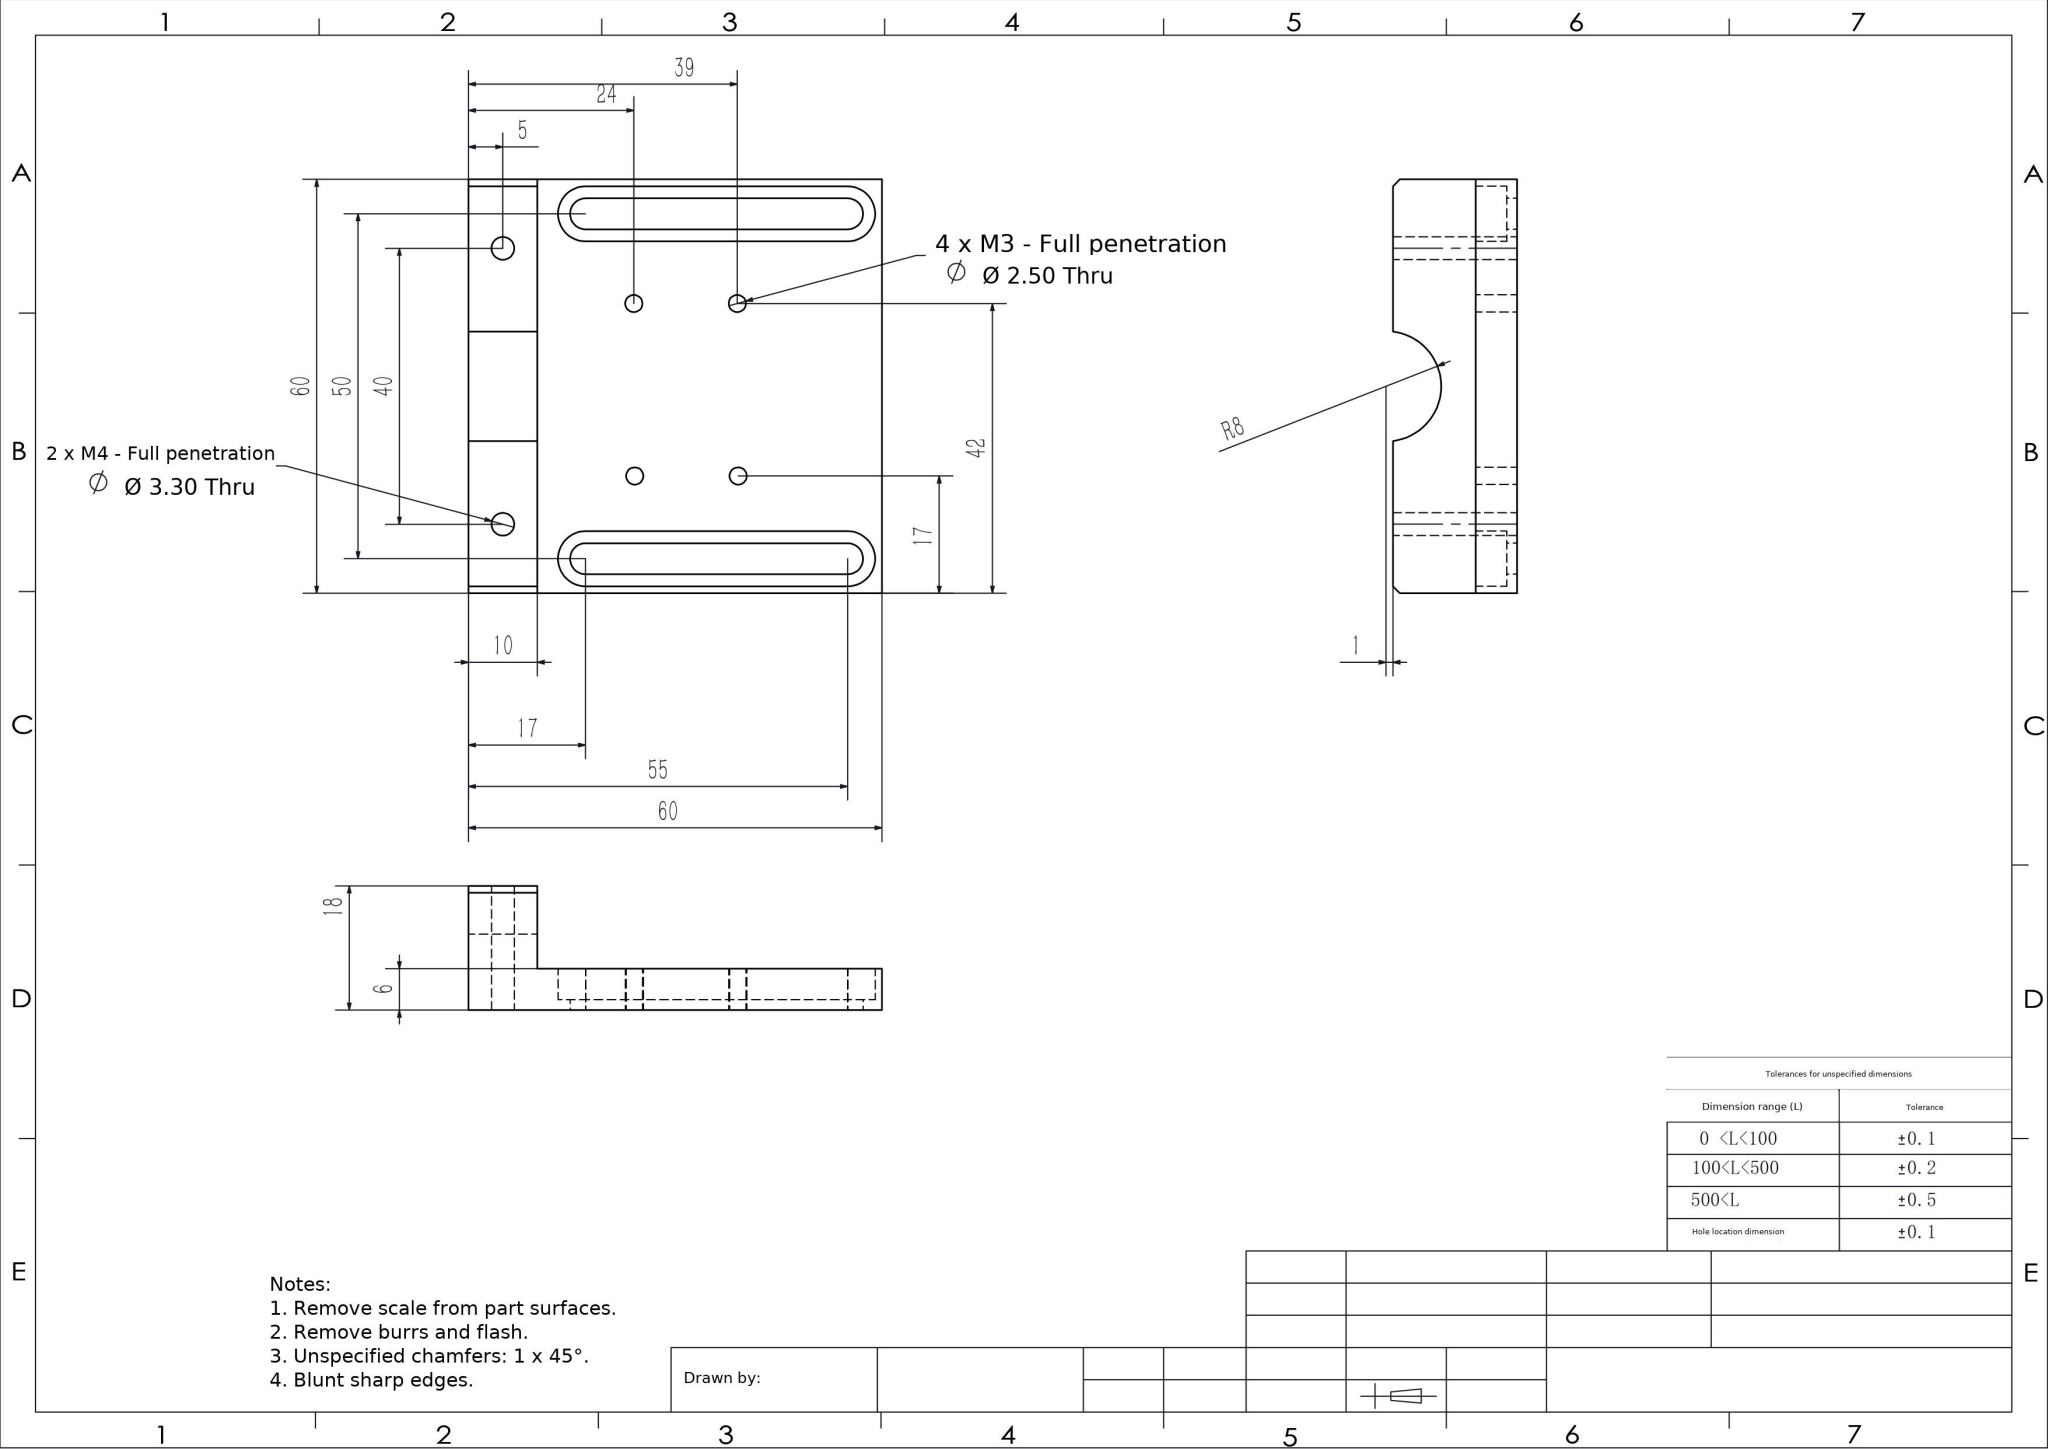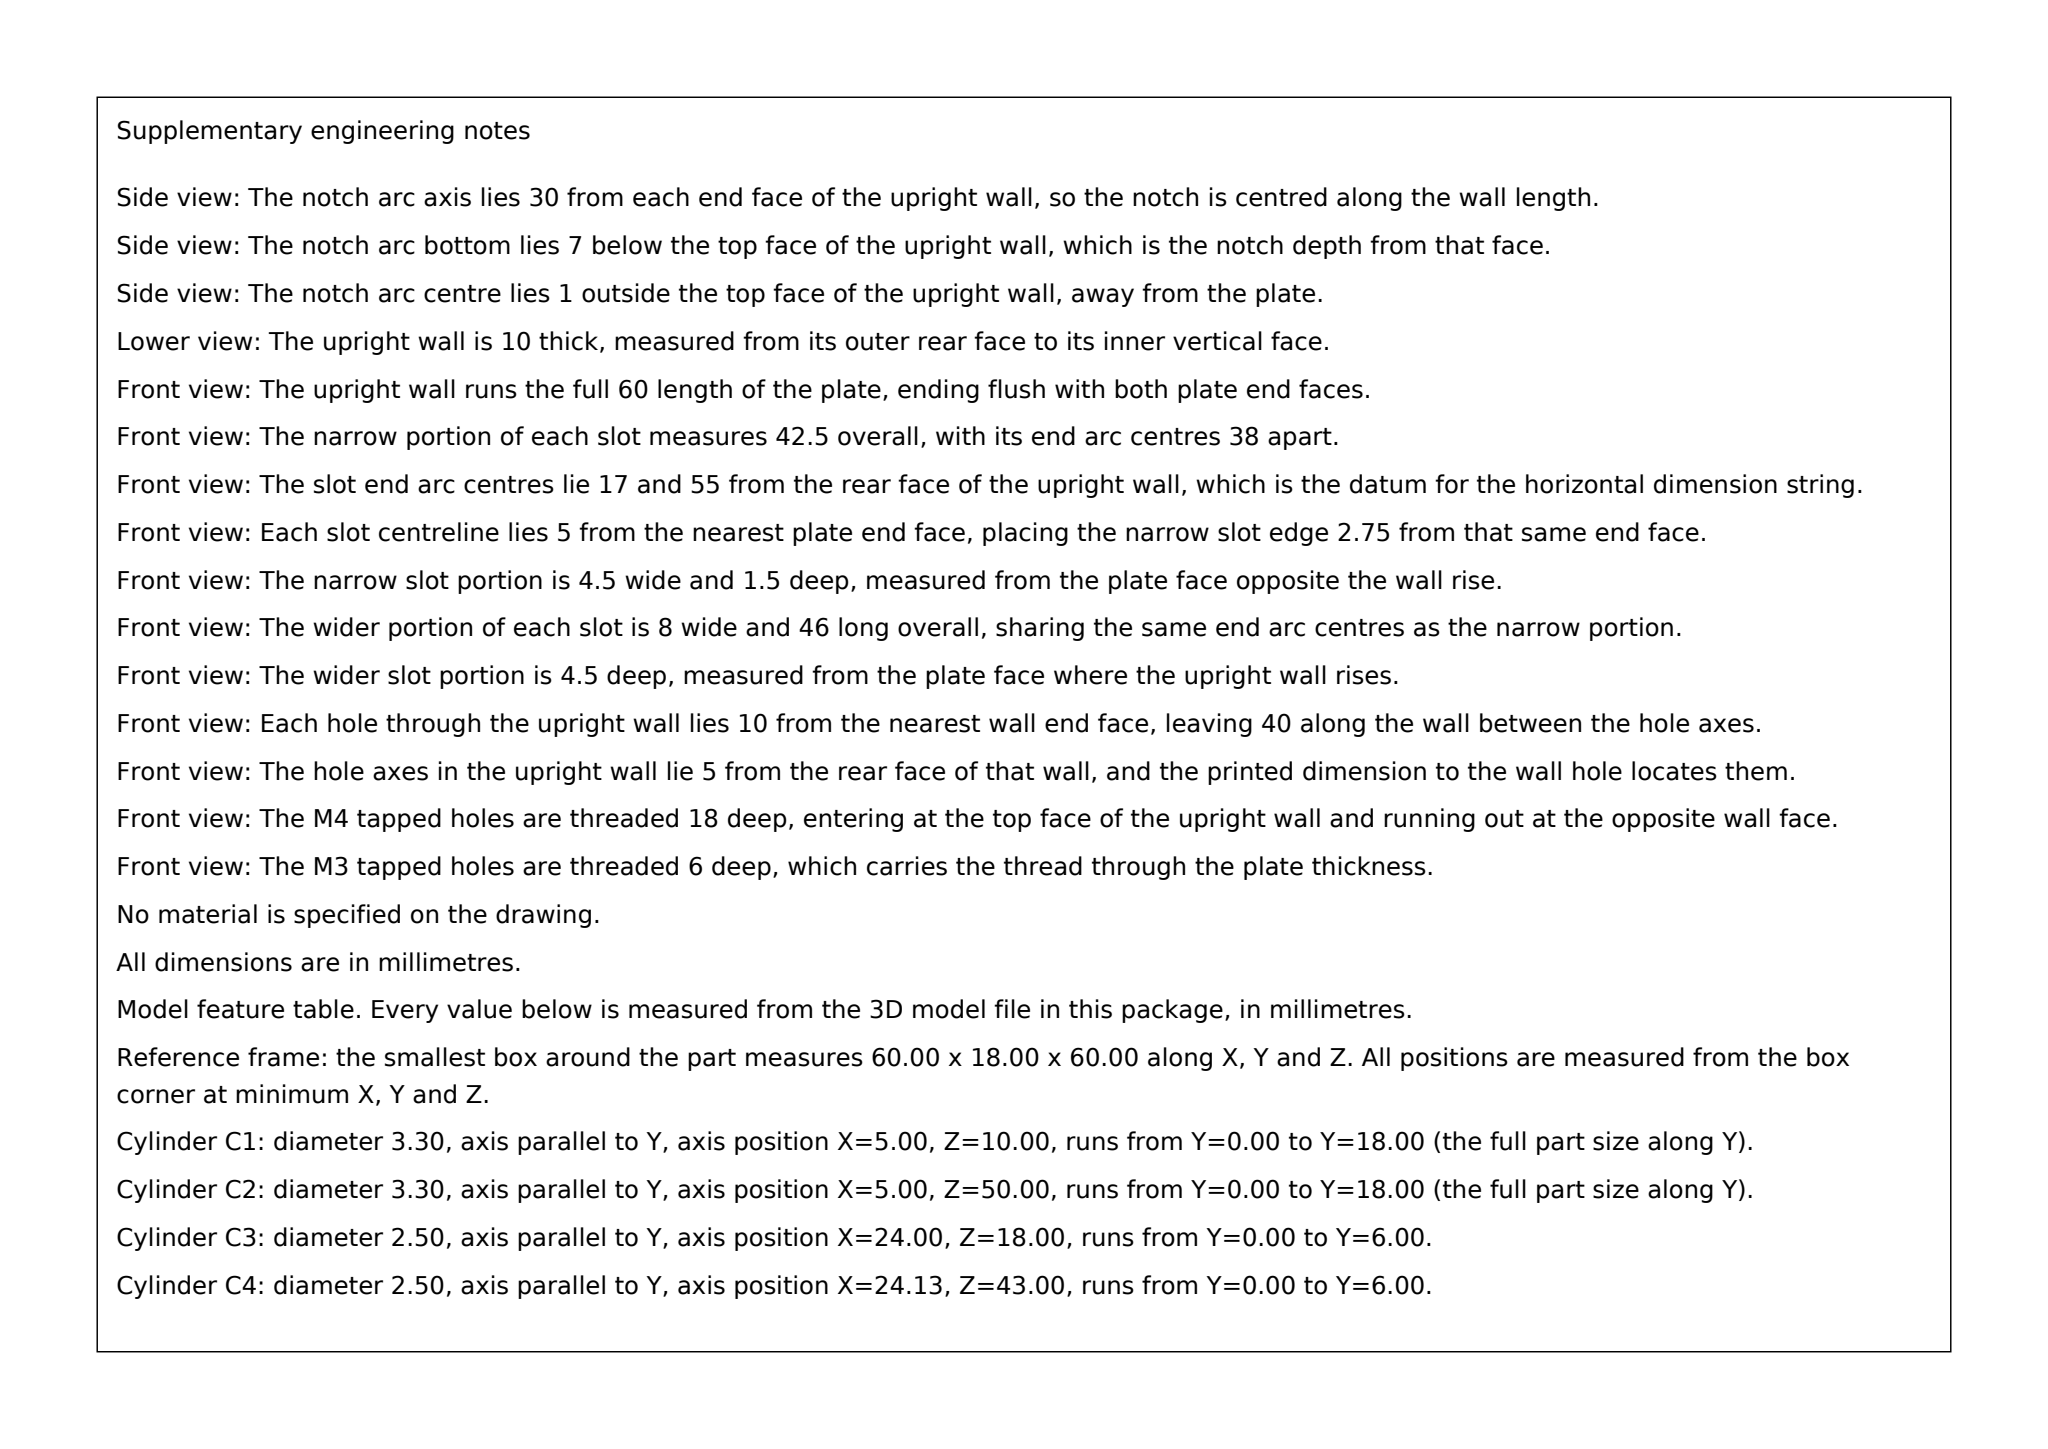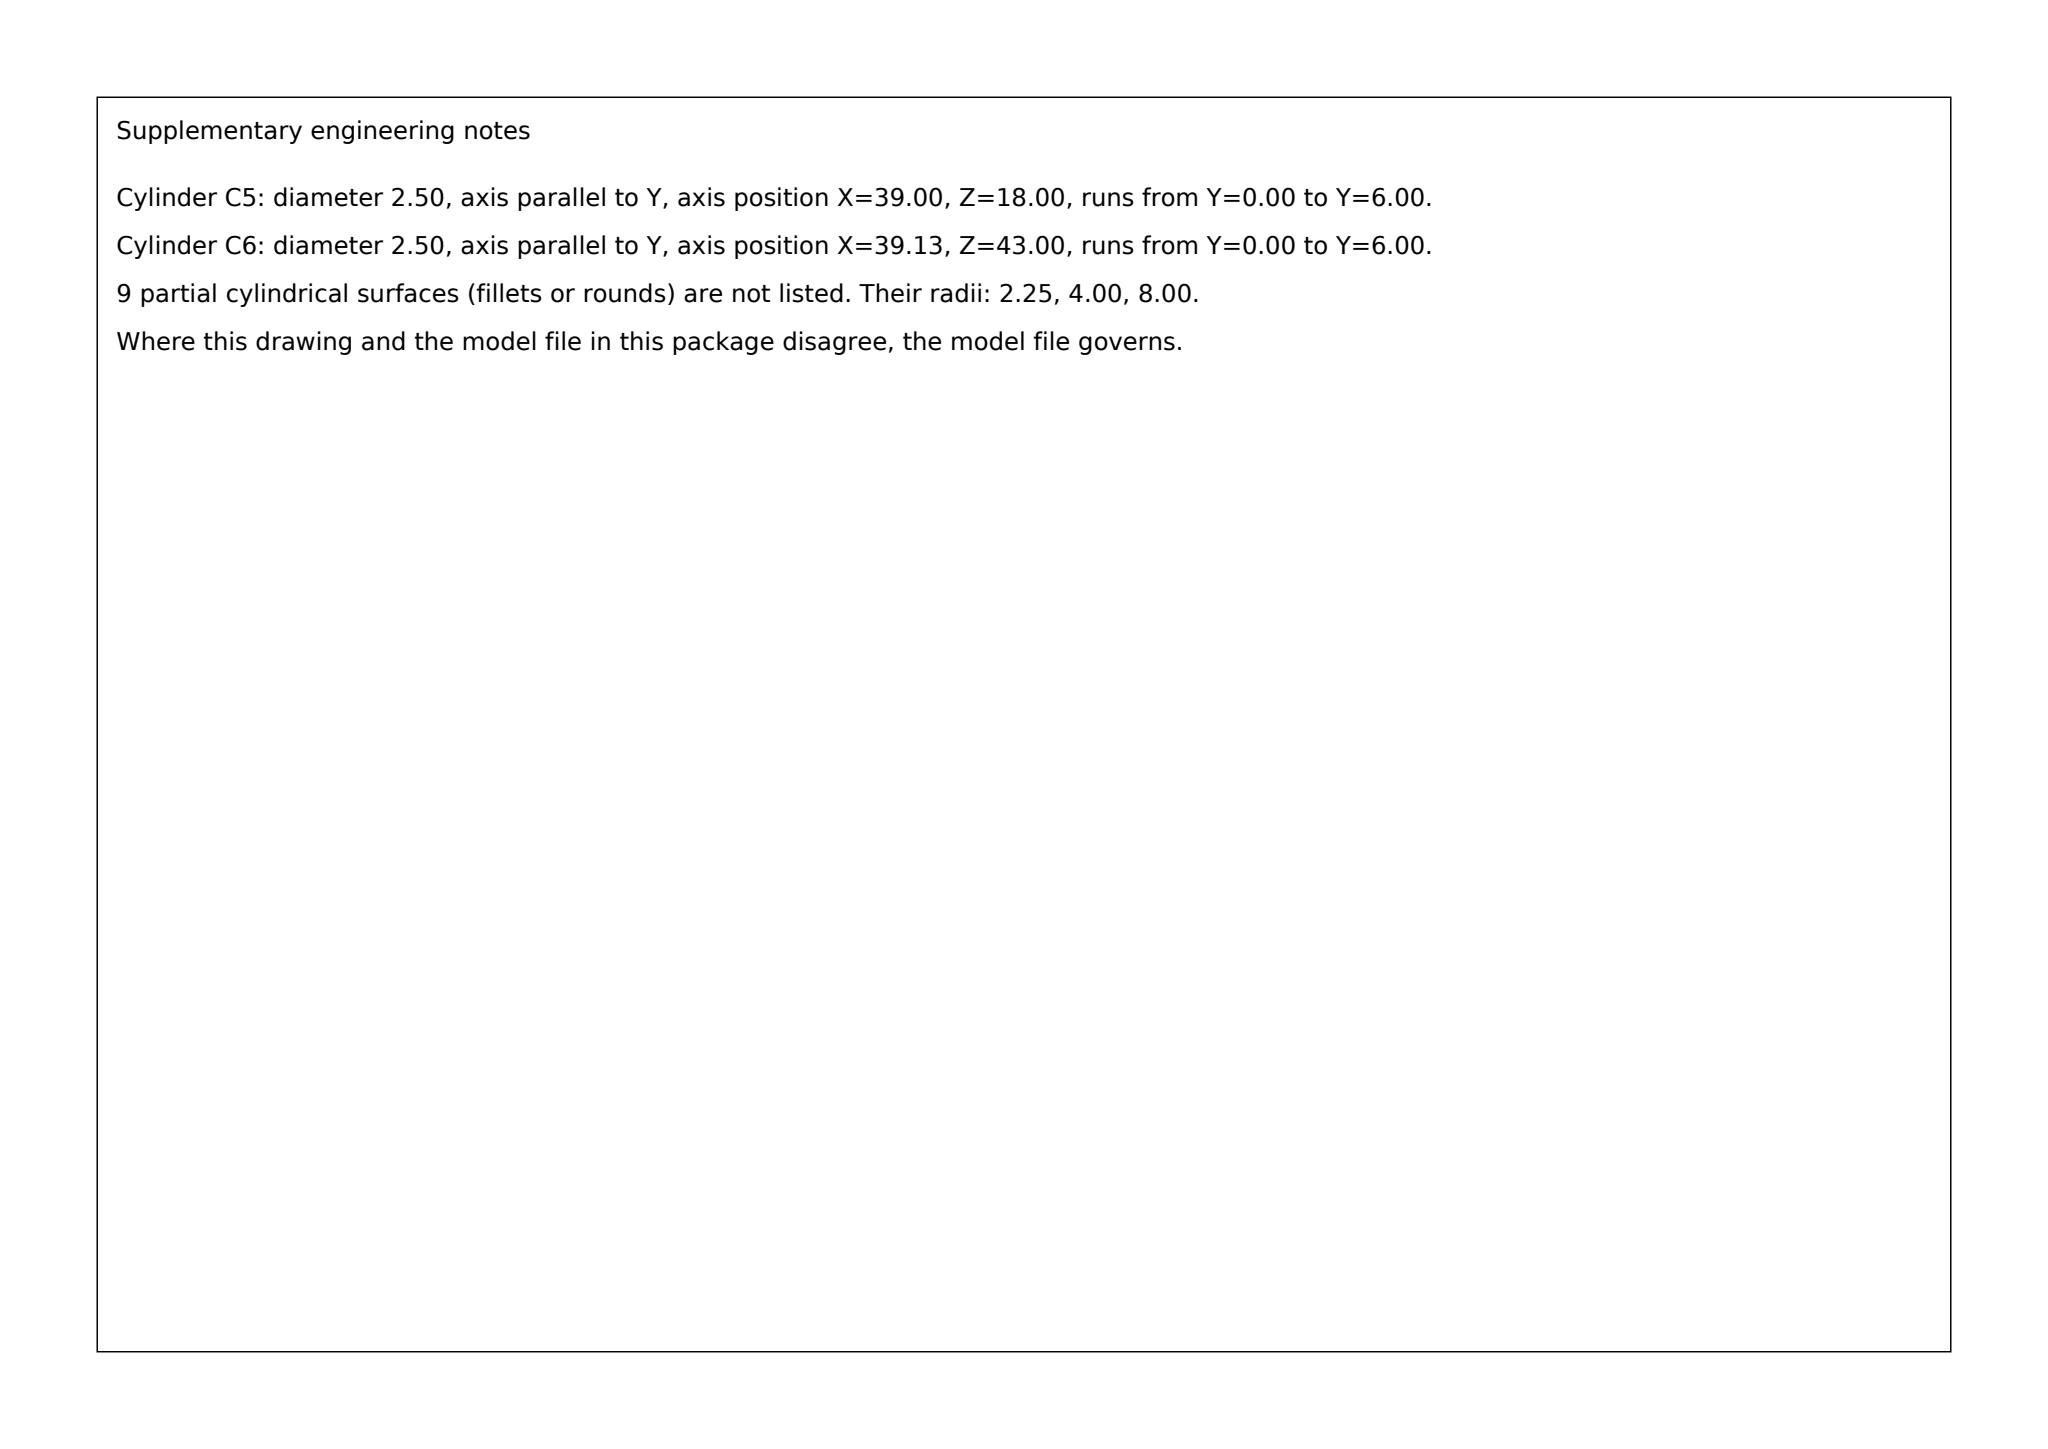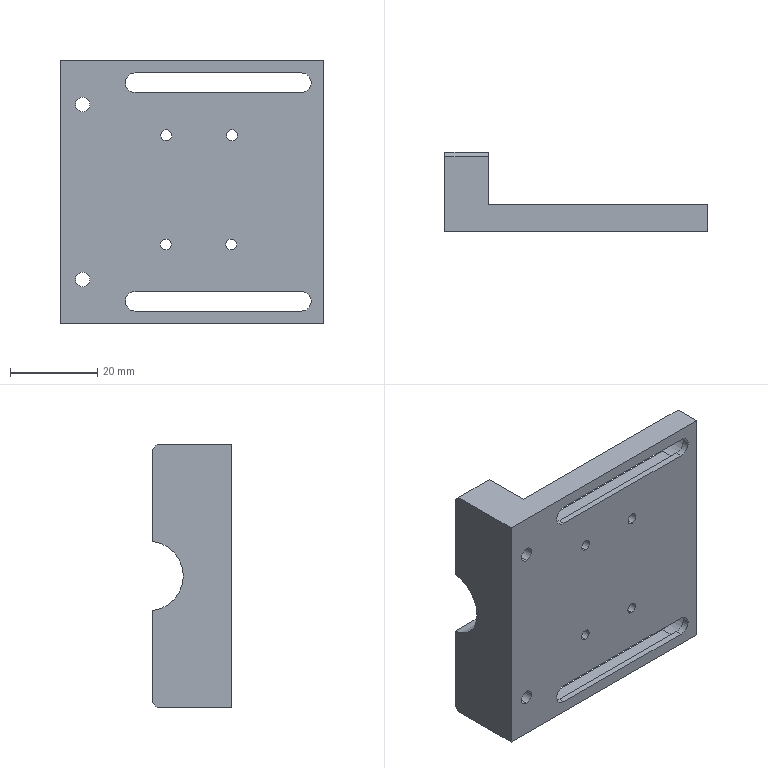Part | SolidWorks | mm | 1 solid | 42 faces | box 60 x 18 x 60 mm | volume 23769 mm3 | cylinder 21 | plane 21 | commonest cylinder face diameters 2.5 x8 3.3 x4 4.5 x4 8 x4 16 x1
build123d program:
from build123d import *

# Parameters (mm, degrees)
BOSS_EXTRUDE1_DEPTH = 60
SKETCH3_R           = 8
CUT_EXTRUDE1_DEPTH  = 81.15
M4_TAPPED_HOLE1_D   = 3.3
CHAMFER1_SIZE       = 1
CUT_EXTRUDE2_DEPTH  = 86.697
CUT_EXTRUDE3_DEPTH  = 4.5
M3_TAPPED_HOLE1_D   = 2.5


with BuildPart() as part:
    # Sketch1 → Boss-Extrude1 (new body)
    with BuildSketch(Plane.XY):
        Polygon((10, 6), (60, 6), (60, 0), (0, 0), (0, 18), (10, 18), align=None)
    extrude(amount=BOSS_EXTRUDE1_DEPTH)

    # Sketch3 → Cut-Extrude1 (cut, through all)
    with BuildSketch(Plane(origin=(10, 0, 0), x_dir=(0, 0, -1), z_dir=(1, 0, 0))):
        with Locations((-30, 19)):
            Circle(SKETCH3_R)
    extrude(amount=-CUT_EXTRUDE1_DEPTH, mode=Mode.SUBTRACT)

    # M4 Tapped Hole1 (through all)
    with Locations(Plane(origin=(0, 18, 0), x_dir=(1, 0, 0), z_dir=(0, 1, 0))):
        with Locations((5, -10), (5, -50)):
            Hole(M4_TAPPED_HOLE1_D / 2)

    # Chamfer1
    chamfer1_edges = [part.edges().sort_by_distance(p)[0] for p in [
        (5, 18, 60),
        (5, 18, 0),
    ]]
    chamfer(chamfer1_edges, length=CHAMFER1_SIZE)

    # Sketch7 → Cut-Extrude2 (cut, through all)
    with BuildSketch(Plane(origin=(0, 6, 0), x_dir=(1, 0, 0), z_dir=(0, 1, 0))):
        with BuildLine():
            Line((17, -52.75), (55, -52.75))
            ThreePointArc((55, -52.75), (57.25, -55), (55, -57.25))
            Line((55, -57.25), (17, -57.25))
            ThreePointArc((17, -57.25), (14.75, -55), (17, -52.75))
        make_face()
        with BuildLine():
            Line((17, -7.25), (55, -7.25))
            ThreePointArc((55, -7.25), (57.25, -5), (55, -2.75))
            Line((55, -2.75), (17, -2.75))
            ThreePointArc((17, -2.75), (14.75, -5), (17, -7.25))
        make_face()
    extrude(amount=-CUT_EXTRUDE2_DEPTH, mode=Mode.SUBTRACT)

    # Sketch8 → Cut-Extrude3 (cut)
    with BuildSketch(Plane(origin=(0, 6, 0), x_dir=(1, 0, 0), z_dir=(0, 1, 0))):
        with BuildLine():
            Line((17, -51), (55, -51))
            ThreePointArc((55, -51), (59, -55), (55, -59))
            Line((55, -59), (17, -59))
            ThreePointArc((17, -59), (13, -55), (17, -51))
        make_face()
        with BuildLine():
            Line((17, -9), (55, -9))
            ThreePointArc((55, -9), (59, -5), (55, -1))
            Line((55, -1), (17, -1))
            ThreePointArc((17, -1), (13, -5), (17, -9))
        make_face()
    extrude(amount=-CUT_EXTRUDE3_DEPTH, mode=Mode.SUBTRACT)

    # M3 Tapped Hole1 (through all)
    with Locations(Plane(origin=(0, 6, 0), x_dir=(1, 0, 0), z_dir=(0, 1, 0))):
        with Locations((39, -18), (24, -18), (39.128, -43), (24.128, -43)):
            Hole(M3_TAPPED_HOLE1_D / 2)


solid = part.part